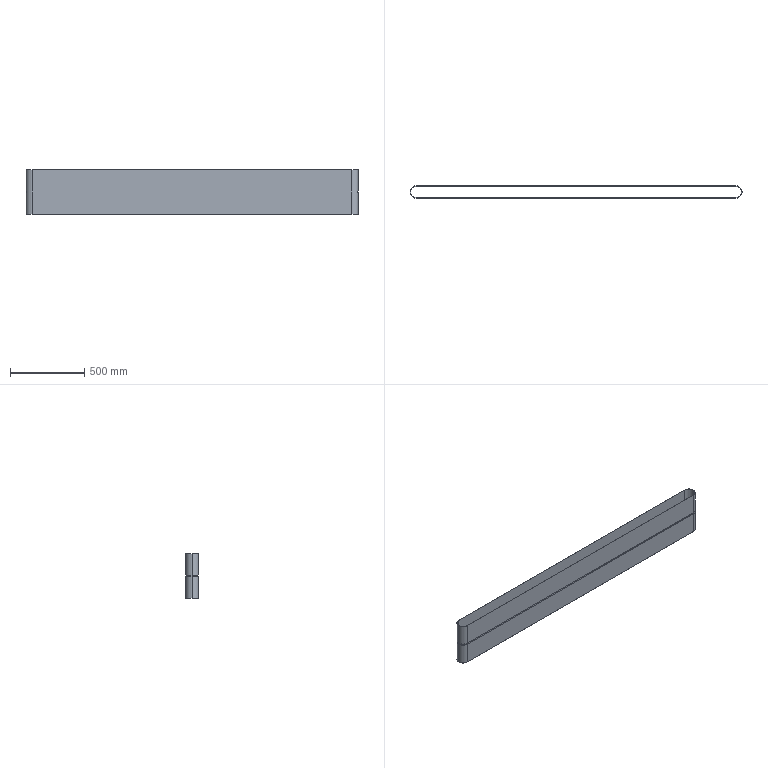Component | SolidWorks | Q1-HBLTDS300-4.55-1 | 1 solid | 52 faces | box 2230.8 x 82.8 x 300 mm | volume 2027073 mm3 | cylinder 22 | plane 18 | cone 8 | torus 4 | commonest cylinder face diameters 80 x8 74 x8 82.8 x4 2 x2
build123d program:
from build123d import *

# Parameters (mm, degrees)
REVOLVE1_ANGLE      = 180
BOSS_EXTRUDE1_DEPTH = 2148
BOSS_EXTRUDE2_DEPTH = 2148


with BuildPart() as part:
    # Sketch1 → Revolve1 (revolve)
    with BuildSketch(Plane(origin=(0, 0, 0), x_dir=(0, 0, -1), z_dir=(1, 0, 0))):
        with BuildLine():
            Line((-300, 41.4), (-300, 40))
            Line((-300, 40), (-155, 40))
            Line((-155, 40), (-153.9, 37))
            Line((-153.9, 37), (-151, 37))
            ThreePointArc((-151, 37), (-150.707, 37.707), (-150, 38))
            Line((-150, 38), (-149, 37))
            Line((-149, 37), (-146.1, 37))
            Line((-146.1, 37), (-145, 40))
            Line((-145, 40), (0, 40))
            Line((0, 40), (0, 41.4))
            Line((0, 41.4), (-300, 41.4))
        make_face()
    revolve1 = revolve(axis=Axis((0, 0, 145), (0, 0, 1)), revolution_arc=REVOLVE1_ANGLE)

    # Sketch2 → Boss-Extrude1 (add)
    with BuildSketch(Plane(origin=(0, 0, 0), x_dir=(0, 0, -1), z_dir=(1, 0, 0))):
        with BuildLine():
            Line((-153.9, 37), (-151, 37))
            ThreePointArc((-151, 37), (-150.707, 37.707), (-150, 38))
            Line((-150, 38), (-149, 37))
            Line((-149, 37), (-146.1, 37))
            Line((-146.1, 37), (-145, 40))
            Line((-145, 40), (0, 40))
            Line((0, 40), (0, 41.4))
            Line((0, 41.4), (-300, 41.4))
            Line((-300, 41.4), (-300, 40))
            Line((-300, 40), (-155, 40))
            Line((-155, 40), (-153.9, 37))
        make_face()
    extrude(amount=BOSS_EXTRUDE1_DEPTH)

    # Sketch4 → Boss-Extrude2 (add)
    with BuildSketch(Plane(origin=(0, 0, 0), x_dir=(0, 0, -1), z_dir=(1, 0, 0))):
        with BuildLine():
            Line((0, -41.4), (0, -40))
            Line((0, -40), (-145, -40))
            Line((-145, -40), (-146.1, -37))
            Line((-146.1, -37), (-149, -37))
            Line((-149, -37), (-150, -38))
            ThreePointArc((-150, -38), (-150.707, -37.707), (-151, -37))
            Line((-151, -37), (-153.9, -37))
            Line((-153.9, -37), (-155, -40))
            Line((-155, -40), (-300, -40))
            Line((-300, -40), (-300, -41.4))
            Line((-300, -41.4), (0, -41.4))
        make_face()
    extrude(amount=BOSS_EXTRUDE2_DEPTH)

    # Mirror1: Revolve1 across plane
    add(revolve1.mirror(Plane(origin=(1074, 0, 0), x_dir=(0, 0, 1), z_dir=(1, 0, 0))))


solid = part.part

# Placed as in the assembly
solid = solid.moved(Location((0, 0, -150), (0, 0, 0)))